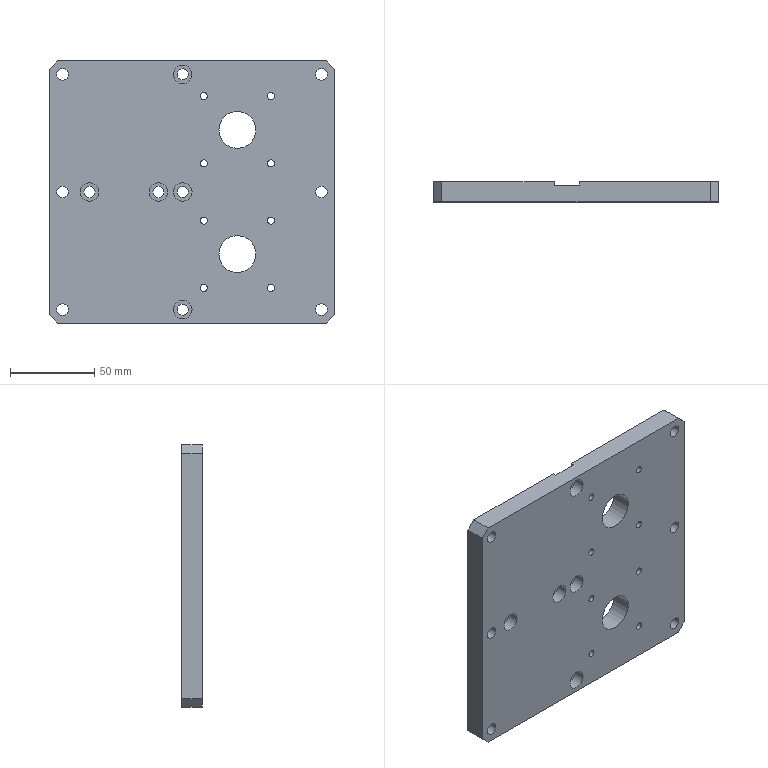Component | SolidWorks | ClampingAssembly-1_A82-1 | 1 solid | 71 faces | box 170 x 12 x 156 mm | volume 295821 mm3 | cylinder 52 | plane 19 | commonest cylinder face diameters 4.2 x16 7 x12 11 x10 6.6 x10 22 x4 | material S45C
build123d program:
from build123d import *

# Parameters (mm, degrees)
SKETCH1_W                                          = 170
SKETCH1_H                                          = 156
BOSS_EXTRUDE1_DEPTH                                = 6
SKETCH2_W                                          = 2
SKETCH2_H                                          = 15
CUT_EXTRUDE1_DEPTH                                 = 178.755
SKETCH3_R                                          = 11
CUT_EXTRUDE2_DEPTH                                 = 116.987
CHAMFER1_SIZE                                      = 5
M5_TAPPED_HOLE1_D                                  = 4.2
HOLE_SIZE_ACCORDING_TO_TYPE_1_OF_HEXAG_D           = 6.6
HOLE_SIZE_ACCORDING_TO_TYPE_1_OF_HEXAG_CBORE_D     = 11
HOLE_SIZE_ACCORDING_TO_TYPE_1_OF_HEXAG_CBORE_DEPTH = 6.8
F_7_0_7_DIAMETER_HOLE1_D                           = 7
HOLE_SIZE_ACCORDING_TO_TYPE_2_OF_HEXAG_D           = 6.6
HOLE_SIZE_ACCORDING_TO_TYPE_2_OF_HEXAG_CBORE_D     = 11
HOLE_SIZE_ACCORDING_TO_TYPE_2_OF_HEXAG_CBORE_DEPTH = 6.8


with BuildPart() as part:
    # Sketch1 → Boss-Extrude1 (new, symmetric)
    with BuildSketch(Plane(origin=(0, 0, 0), x_dir=(0, 0, -1), z_dir=(1, 0, 0))):
        Rectangle(SKETCH1_W, SKETCH1_H)
    extrude(amount=BOSS_EXTRUDE1_DEPTH, both=True)

    # Sketch2 → Cut-Extrude1 (cut, through all)
    with BuildSketch(Plane.XZ.offset(78)):
        with Locations((5, 5.5)):
            Rectangle(SKETCH2_W, SKETCH2_H)
    extrude(amount=-CUT_EXTRUDE1_DEPTH, mode=Mode.SUBTRACT)

    # Sketch3 → Cut-Extrude2 (cut, through all)
    with BuildSketch(Plane(origin=(6, 0, 0), x_dir=(0, 0, -1), z_dir=(1, 0, 0))):
        with Locations((27, 37)):
            Circle(SKETCH3_R)
    cut_extrude2 = extrude(amount=-CUT_EXTRUDE2_DEPTH, mode=Mode.SUBTRACT)

    # Chamfer1
    chamfer1_edges = [part.edges().sort_by_distance(p)[0] for p in [
        (0, -78, -85),
        (0, -78, 85),
        (0, 78, 85),
        (0, 78, -85),
    ]]
    chamfer(chamfer1_edges, length=CHAMFER1_SIZE)

    # M5 Tapped Hole1 (through all)
    with Locations(Plane(origin=(6, 0, 0), x_dir=(0, 0, -1), z_dir=(1, 0, 0))):
        with Locations((7, 57), (47, 57), (47, 17), (7, 17)):
            m5_tapped_hole1 = Hole(M5_TAPPED_HOLE1_D / 2)

    # Hole Size _According to_ Type 1 of Hexag (through all)
    with Locations(Plane.ZY.offset(6)):
        with Locations((20, 0), (61, 0)):
            CounterBoreHole(HOLE_SIZE_ACCORDING_TO_TYPE_1_OF_HEXAG_D / 2, HOLE_SIZE_ACCORDING_TO_TYPE_1_OF_HEXAG_CBORE_D / 2, HOLE_SIZE_ACCORDING_TO_TYPE_1_OF_HEXAG_CBORE_DEPTH)

    # 7.0 _7_ Diameter Hole1 (through all)
    with Locations(Plane(origin=(6, 0, 0), x_dir=(0, 0, -1), z_dir=(1, 0, 0))):
        with Locations((-77, 70), (-77, -70), (77, -70), (77, 70), (-77, 0), (77, 0)):
            Hole(F_7_0_7_DIAMETER_HOLE1_D / 2)

    # Mirror1: Cut-Extrude2, M5 Tapped Hole1 across plane
    add(cut_extrude2.mirror(Plane.ZX), mode=Mode.SUBTRACT)
    add(m5_tapped_hole1.mirror(Plane.ZX), mode=Mode.SUBTRACT)

    # Hole Size _According to_ Type 2 of Hexag (through all)
    with Locations(Plane.ZY.offset(6)):
        with Locations((5.5, -70), (5.5, 0), (5.5, 70)):
            CounterBoreHole(HOLE_SIZE_ACCORDING_TO_TYPE_2_OF_HEXAG_D / 2, HOLE_SIZE_ACCORDING_TO_TYPE_2_OF_HEXAG_CBORE_D / 2, HOLE_SIZE_ACCORDING_TO_TYPE_2_OF_HEXAG_CBORE_DEPTH)


solid = part.part

# Placed as in the assembly
solid = solid.moved(Location((-16.551, -29.964, -0.5), (-90, -90, 0)))